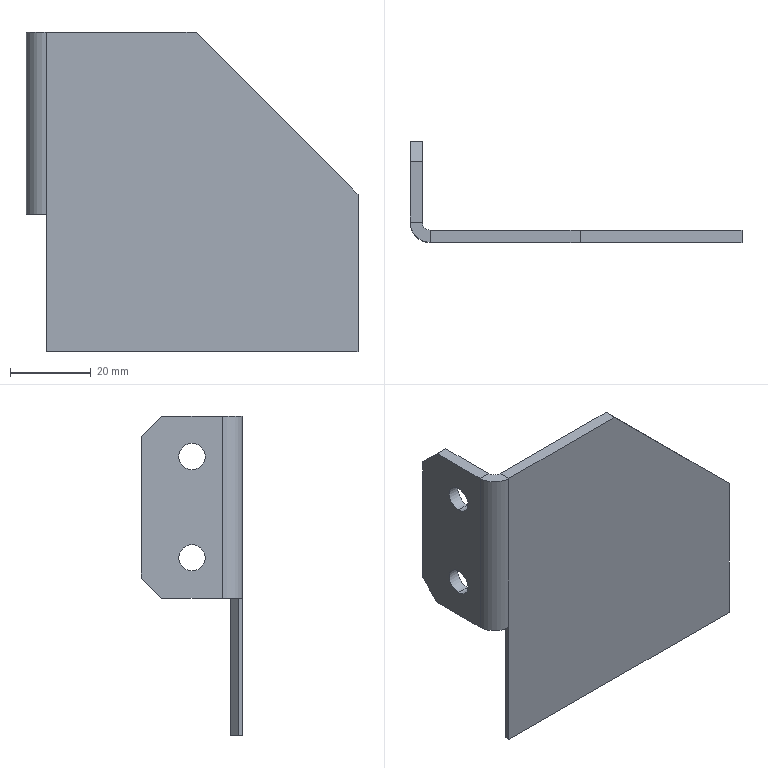Component | SolidWorks | OPW-05-033-1 | 1 solid | 22 faces | box 82 x 25 x 79 mm | volume 18949 mm3 | plane 16 | cylinder 6 | commonest cylinder face diameters 6.5 x4 4 x1 10 x1
STEP:
#1=COLOUR_RGB('',0.7922,0.8196,0.9333);
#2=FILL_AREA_STYLE_COLOUR('',#1);
#3=FILL_AREA_STYLE('',(#2));
#4=SURFACE_STYLE_FILL_AREA(#3);
#5=SURFACE_SIDE_STYLE('',(#4));
#6=SURFACE_STYLE_USAGE(.BOTH.,#5);
#7=PRESENTATION_STYLE_ASSIGNMENT((#6));
#8=CARTESIAN_POINT('',(1.775,9.035,0.9154));
#9=VERTEX_POINT('',#8);
#10=CARTESIAN_POINT('',(1.775,9.035,0.6594));
#11=VERTEX_POINT('',#10);
#12=CARTESIAN_POINT('',(1.775,9.035,0.7874));
#13=DIRECTION('',(1.,-0.,0.));
#14=DIRECTION('',(0.,1.,0.));
#15=AXIS2_PLACEMENT_3D('',#12,#13,#14);
#16=CIRCLE('',#15,0.128);
#17=EDGE_CURVE('',#9,#11,#16,.T.);
#18=ORIENTED_EDGE('',*,*,#17,.F.);
#19=CARTESIAN_POINT('',(1.894,9.035,0.9154));
#20=VERTEX_POINT('',#19);
#21=CARTESIAN_POINT('',(1.894,9.035,0.9154));
#22=DIRECTION('',(1.,0.,0.));
#23=VECTOR('',#22,39.37);
#24=LINE('',#21,#23);
#25=EDGE_CURVE('',#9,#20,#24,.T.);
#26=ORIENTED_EDGE('',*,*,#25,.T.);
#27=CARTESIAN_POINT('',(1.894,9.035,0.6594));
#28=VERTEX_POINT('',#27);
#29=CARTESIAN_POINT('',(1.894,9.035,0.7874));
#30=DIRECTION('',(1.,0.,0.));
#31=DIRECTION('',(0.,0.,-1.));
#32=AXIS2_PLACEMENT_3D('',#29,#30,#31);
#33=CIRCLE('',#32,0.128);
#34=EDGE_CURVE('',#20,#28,#33,.T.);
#35=ORIENTED_EDGE('',*,*,#34,.T.);
#36=CARTESIAN_POINT('',(1.894,9.035,0.6594));
#37=DIRECTION('',(1.,0.,0.));
#38=VECTOR('',#37,39.37);
#39=LINE('',#36,#38);
#40=EDGE_CURVE('',#11,#28,#39,.T.);
#41=ORIENTED_EDGE('',*,*,#40,.F.);
#42=EDGE_LOOP('',(#18,#26,#35,#41));
#43=FACE_OUTER_BOUND('',#42,.T.);
#44=CARTESIAN_POINT('',(1.894,9.035,0.7874));
#45=DIRECTION('',(1.,0.,0.));
#46=DIRECTION('',(0.,0.,-1.));
#47=AXIS2_PLACEMENT_3D('',#44,#45,#46);
#48=CYLINDRICAL_SURFACE('',#47,0.128);
#49=ADVANCED_FACE('',(#43),#48,.F.);
#50=CARTESIAN_POINT('',(1.775,9.035,-0.0689));
#51=VERTEX_POINT('',#50);
#52=CARTESIAN_POINT('',(1.775,9.035,-0.3248));
#53=VERTEX_POINT('',#52);
#54=CARTESIAN_POINT('',(1.775,9.035,-0.1969));
#55=DIRECTION('',(1.,-0.,0.));
#56=DIRECTION('',(0.,1.,0.));
#57=AXIS2_PLACEMENT_3D('',#54,#55,#56);
#58=CIRCLE('',#57,0.128);
#59=EDGE_CURVE('',#51,#53,#58,.T.);
#60=ORIENTED_EDGE('',*,*,#59,.F.);
#61=CARTESIAN_POINT('',(1.894,9.035,-0.0689));
#62=VERTEX_POINT('',#61);
#63=CARTESIAN_POINT('',(1.894,9.035,-0.0689));
#64=DIRECTION('',(1.,0.,0.));
#65=VECTOR('',#64,39.37);
#66=LINE('',#63,#65);
#67=EDGE_CURVE('',#51,#62,#66,.T.);
#68=ORIENTED_EDGE('',*,*,#67,.T.);
#69=CARTESIAN_POINT('',(1.894,9.035,-0.3248));
#70=VERTEX_POINT('',#69);
#71=CARTESIAN_POINT('',(1.894,9.035,-0.1969));
#72=DIRECTION('',(1.,0.,0.));
#73=DIRECTION('',(0.,0.,-1.));
#74=AXIS2_PLACEMENT_3D('',#71,#72,#73);
#75=CIRCLE('',#74,0.128);
#76=EDGE_CURVE('',#62,#70,#75,.T.);
#77=ORIENTED_EDGE('',*,*,#76,.T.);
#78=CARTESIAN_POINT('',(1.894,9.035,-0.3248));
#79=DIRECTION('',(1.,0.,0.));
#80=VECTOR('',#79,39.37);
#81=LINE('',#78,#80);
#82=EDGE_CURVE('',#53,#70,#81,.T.);
#83=ORIENTED_EDGE('',*,*,#82,.F.);
#84=EDGE_LOOP('',(#60,#68,#77,#83));
#85=FACE_OUTER_BOUND('',#84,.T.);
#86=CARTESIAN_POINT('',(1.894,9.035,-0.1969));
#87=DIRECTION('',(1.,0.,0.));
#88=DIRECTION('',(0.,0.,-1.));
#89=AXIS2_PLACEMENT_3D('',#86,#87,#88);
#90=CYLINDRICAL_SURFACE('',#89,0.128);
#91=ADVANCED_FACE('',(#85),#90,.F.);
#92=CARTESIAN_POINT('',(1.775,8.74,1.181));
#93=VERTEX_POINT('',#92);
#94=CARTESIAN_POINT('',(1.894,8.74,1.181));
#95=VERTEX_POINT('',#94);
#96=CARTESIAN_POINT('',(1.775,8.74,1.181));
#97=DIRECTION('',(1.,0.,0.));
#98=VECTOR('',#97,39.37);
#99=LINE('',#96,#98);
#100=EDGE_CURVE('',#93,#95,#99,.T.);
#101=ORIENTED_EDGE('',*,*,#100,.F.);
#102=CARTESIAN_POINT('',(1.972,8.543,1.181));
#103=VERTEX_POINT('',#102);
#104=CARTESIAN_POINT('',(1.972,8.74,1.181));
#105=DIRECTION('',(0.,0.,1.));
#106=DIRECTION('',(-1.,0.,0.));
#107=AXIS2_PLACEMENT_3D('',#104,#105,#106);
#108=CIRCLE('',#107,0.1969);
#109=EDGE_CURVE('',#93,#103,#108,.T.);
#110=ORIENTED_EDGE('',*,*,#109,.T.);
#111=CARTESIAN_POINT('',(1.972,8.661,1.181));
#112=VERTEX_POINT('',#111);
#113=CARTESIAN_POINT('',(1.972,8.661,1.181));
#114=DIRECTION('',(0.,-1.,0.));
#115=VECTOR('',#114,39.37);
#116=LINE('',#113,#115);
#117=EDGE_CURVE('',#112,#103,#116,.T.);
#118=ORIENTED_EDGE('',*,*,#117,.F.);
#119=CARTESIAN_POINT('',(1.972,8.74,1.181));
#120=DIRECTION('',(0.,0.,1.));
#121=DIRECTION('',(1.,0.,0.));
#122=AXIS2_PLACEMENT_3D('',#119,#120,#121);
#123=CIRCLE('',#122,0.07874);
#124=EDGE_CURVE('',#95,#112,#123,.T.);
#125=ORIENTED_EDGE('',*,*,#124,.F.);
#126=EDGE_LOOP('',(#101,#110,#118,#125));
#127=FACE_OUTER_BOUND('',#126,.T.);
#128=CARTESIAN_POINT('',(1.775,8.74,1.181));
#129=DIRECTION('',(0.,0.,1.));
#130=DIRECTION('',(1.,0.,0.));
#131=AXIS2_PLACEMENT_3D('',#128,#129,#130);
#132=PLANE('',#131);
#133=ADVANCED_FACE('',(#127),#132,.T.);
#134=CARTESIAN_POINT('',(1.894,9.331,1.181));
#135=VERTEX_POINT('',#134);
#136=CARTESIAN_POINT('',(1.894,9.528,1.181));
#137=DIRECTION('',(-0.,-1.,0.));
#138=VECTOR('',#137,39.37);
#139=LINE('',#136,#138);
#140=EDGE_CURVE('',#135,#95,#139,.T.);
#141=ORIENTED_EDGE('',*,*,#140,.F.);
#142=CARTESIAN_POINT('',(1.775,9.331,1.181));
#143=VERTEX_POINT('',#142);
#144=CARTESIAN_POINT('',(1.972,9.331,1.181));
#145=DIRECTION('',(-1.,0.,0.));
#146=VECTOR('',#145,39.37);
#147=LINE('',#144,#146);
#148=EDGE_CURVE('',#135,#143,#147,.T.);
#149=ORIENTED_EDGE('',*,*,#148,.T.);
#150=CARTESIAN_POINT('',(1.775,9.528,1.181));
#151=DIRECTION('',(-0.,-1.,0.));
#152=VECTOR('',#151,39.37);
#153=LINE('',#150,#152);
#154=EDGE_CURVE('',#143,#93,#153,.T.);
#155=ORIENTED_EDGE('',*,*,#154,.T.);
#156=ORIENTED_EDGE('',*,*,#100,.T.);
#157=EDGE_LOOP('',(#141,#149,#155,#156));
#158=FACE_OUTER_BOUND('',#157,.T.);
#159=CARTESIAN_POINT('',(1.972,8.661,1.181));
#160=DIRECTION('',(0.,0.,1.));
#161=DIRECTION('',(1.,0.,0.));
#162=AXIS2_PLACEMENT_3D('',#159,#160,#161);
#163=PLANE('',#162);
#164=ADVANCED_FACE('',(#158),#163,.T.);
#165=CARTESIAN_POINT('',(1.972,8.543,-1.929));
#166=VERTEX_POINT('',#165);
#167=CARTESIAN_POINT('',(1.972,8.583,-1.929));
#168=VERTEX_POINT('',#167);
#169=CARTESIAN_POINT('',(1.972,8.543,-1.929));
#170=DIRECTION('',(0.,1.,0.));
#171=VECTOR('',#170,39.37);
#172=LINE('',#169,#171);
#173=EDGE_CURVE('',#166,#168,#172,.T.);
#174=ORIENTED_EDGE('',*,*,#173,.T.);
#175=CARTESIAN_POINT('',(2.051,8.661,-1.929));
#176=VERTEX_POINT('',#175);
#177=CARTESIAN_POINT('',(2.012,8.622,-1.929));
#178=DIRECTION('',(0.7071,0.7071,0.));
#179=VECTOR('',#178,39.37);
#180=LINE('',#177,#179);
#181=EDGE_CURVE('',#168,#176,#180,.T.);
#182=ORIENTED_EDGE('',*,*,#181,.T.);
#183=CARTESIAN_POINT('',(5.004,8.661,-1.929));
#184=VERTEX_POINT('',#183);
#185=CARTESIAN_POINT('',(1.775,8.661,-1.929));
#186=DIRECTION('',(1.,0.,0.));
#187=VECTOR('',#186,39.37);
#188=LINE('',#185,#187);
#189=EDGE_CURVE('',#176,#184,#188,.T.);
#190=ORIENTED_EDGE('',*,*,#189,.T.);
#191=CARTESIAN_POINT('',(5.004,8.543,-1.929));
#192=VERTEX_POINT('',#191);
#193=CARTESIAN_POINT('',(5.004,8.661,-1.929));
#194=DIRECTION('',(0.,-1.,0.));
#195=VECTOR('',#194,39.37);
#196=LINE('',#193,#195);
#197=EDGE_CURVE('',#184,#192,#196,.T.);
#198=ORIENTED_EDGE('',*,*,#197,.T.);
#199=CARTESIAN_POINT('',(1.775,8.543,-1.929));
#200=DIRECTION('',(1.,0.,0.));
#201=VECTOR('',#200,39.37);
#202=LINE('',#199,#201);
#203=EDGE_CURVE('',#166,#192,#202,.T.);
#204=ORIENTED_EDGE('',*,*,#203,.F.);
#205=EDGE_LOOP('',(#174,#182,#190,#198,#204));
#206=FACE_OUTER_BOUND('',#205,.T.);
#207=CARTESIAN_POINT('',(1.894,8.74,-1.929));
#208=DIRECTION('',(0.,0.,-1.));
#209=DIRECTION('',(-1.,0.,0.));
#210=AXIS2_PLACEMENT_3D('',#207,#208,#209);
#211=PLANE('',#210);
#212=ADVANCED_FACE('',(#206),#211,.T.);
#213=CARTESIAN_POINT('',(5.004,8.543,-0.3937));
#214=VERTEX_POINT('',#213);
#215=CARTESIAN_POINT('',(5.004,8.543,1.181));
#216=DIRECTION('',(0.,0.,-1.));
#217=VECTOR('',#216,39.37);
#218=LINE('',#215,#217);
#219=EDGE_CURVE('',#214,#192,#218,.T.);
#220=ORIENTED_EDGE('',*,*,#219,.F.);
#221=CARTESIAN_POINT('',(3.429,8.543,1.181));
#222=VERTEX_POINT('',#221);
#223=CARTESIAN_POINT('',(5.004,8.543,-0.3937));
#224=DIRECTION('',(-0.7071,0.,0.7071));
#225=VECTOR('',#224,39.37);
#226=LINE('',#223,#225);
#227=EDGE_CURVE('',#214,#222,#226,.T.);
#228=ORIENTED_EDGE('',*,*,#227,.T.);
#229=CARTESIAN_POINT('',(1.775,8.543,1.181));
#230=DIRECTION('',(1.,0.,0.));
#231=VECTOR('',#230,39.37);
#232=LINE('',#229,#231);
#233=EDGE_CURVE('',#103,#222,#232,.T.);
#234=ORIENTED_EDGE('',*,*,#233,.F.);
#235=CARTESIAN_POINT('',(1.972,8.543,-0.5906));
#236=VERTEX_POINT('',#235);
#237=CARTESIAN_POINT('',(1.972,8.543,1.181));
#238=DIRECTION('',(0.,0.,-1.));
#239=VECTOR('',#238,39.37);
#240=LINE('',#237,#239);
#241=EDGE_CURVE('',#103,#236,#240,.T.);
#242=ORIENTED_EDGE('',*,*,#241,.T.);
#243=CARTESIAN_POINT('',(1.972,8.543,-1.929));
#244=DIRECTION('',(-0.,0.,-1.));
#245=VECTOR('',#244,39.37);
#246=LINE('',#243,#245);
#247=EDGE_CURVE('',#236,#166,#246,.T.);
#248=ORIENTED_EDGE('',*,*,#247,.T.);
#249=ORIENTED_EDGE('',*,*,#203,.T.);
#250=EDGE_LOOP('',(#220,#228,#234,#242,#248,#249));
#251=FACE_OUTER_BOUND('',#250,.T.);
#252=CARTESIAN_POINT('',(1.775,8.543,1.181));
#253=DIRECTION('',(0.,1.,0.));
#254=DIRECTION('',(0.,0.,1.));
#255=AXIS2_PLACEMENT_3D('',#252,#253,#254);
#256=PLANE('',#255);
#257=ADVANCED_FACE('',(#251),#256,.F.);
#258=CARTESIAN_POINT('',(5.004,8.661,-0.3937));
#259=VERTEX_POINT('',#258);
#260=CARTESIAN_POINT('',(5.004,8.661,1.181));
#261=DIRECTION('',(0.,0.,-1.));
#262=VECTOR('',#261,39.37);
#263=LINE('',#260,#262);
#264=EDGE_CURVE('',#259,#184,#263,.T.);
#265=ORIENTED_EDGE('',*,*,#264,.F.);
#266=CARTESIAN_POINT('',(5.004,8.661,-0.3937));
#267=DIRECTION('',(0.,-1.,0.));
#268=VECTOR('',#267,39.37);
#269=LINE('',#266,#268);
#270=EDGE_CURVE('',#259,#214,#269,.T.);
#271=ORIENTED_EDGE('',*,*,#270,.T.);
#272=ORIENTED_EDGE('',*,*,#219,.T.);
#273=ORIENTED_EDGE('',*,*,#197,.F.);
#274=EDGE_LOOP('',(#265,#271,#272,#273));
#275=FACE_OUTER_BOUND('',#274,.T.);
#276=CARTESIAN_POINT('',(5.004,8.661,1.181));
#277=DIRECTION('',(1.,0.,0.));
#278=DIRECTION('',(0.,0.,-1.));
#279=AXIS2_PLACEMENT_3D('',#276,#277,#278);
#280=PLANE('',#279);
#281=ADVANCED_FACE('',(#275),#280,.T.);
#282=CARTESIAN_POINT('',(3.429,8.661,1.181));
#283=VERTEX_POINT('',#282);
#284=CARTESIAN_POINT('',(1.775,8.661,1.181));
#285=DIRECTION('',(1.,0.,0.));
#286=VECTOR('',#285,39.37);
#287=LINE('',#284,#286);
#288=EDGE_CURVE('',#112,#283,#287,.T.);
#289=ORIENTED_EDGE('',*,*,#288,.T.);
#290=CARTESIAN_POINT('',(2.602,8.661,2.008));
#291=DIRECTION('',(0.7071,0.,-0.7071));
#292=VECTOR('',#291,39.37);
#293=LINE('',#290,#292);
#294=EDGE_CURVE('',#283,#259,#293,.T.);
#295=ORIENTED_EDGE('',*,*,#294,.T.);
#296=ORIENTED_EDGE('',*,*,#264,.T.);
#297=ORIENTED_EDGE('',*,*,#189,.F.);
#298=CARTESIAN_POINT('',(2.051,8.661,-0.5906));
#299=VERTEX_POINT('',#298);
#300=CARTESIAN_POINT('',(2.051,8.661,-0.5906));
#301=DIRECTION('',(0.,0.,1.));
#302=VECTOR('',#301,39.37);
#303=LINE('',#300,#302);
#304=EDGE_CURVE('',#176,#299,#303,.T.);
#305=ORIENTED_EDGE('',*,*,#304,.T.);
#306=CARTESIAN_POINT('',(1.972,8.661,-0.5906));
#307=VERTEX_POINT('',#306);
#308=CARTESIAN_POINT('',(1.775,8.661,-0.5906));
#309=DIRECTION('',(-1.,0.,0.));
#310=VECTOR('',#309,39.37);
#311=LINE('',#308,#310);
#312=EDGE_CURVE('',#299,#307,#311,.T.);
#313=ORIENTED_EDGE('',*,*,#312,.T.);
#314=CARTESIAN_POINT('',(1.972,8.661,1.181));
#315=DIRECTION('',(0.,0.,-1.));
#316=VECTOR('',#315,39.37);
#317=LINE('',#314,#316);
#318=EDGE_CURVE('',#112,#307,#317,.T.);
#319=ORIENTED_EDGE('',*,*,#318,.F.);
#320=EDGE_LOOP('',(#289,#295,#296,#297,#305,#313,#319));
#321=FACE_OUTER_BOUND('',#320,.T.);
#322=CARTESIAN_POINT('',(1.775,8.661,1.181));
#323=DIRECTION('',(0.,1.,0.));
#324=DIRECTION('',(0.,0.,1.));
#325=AXIS2_PLACEMENT_3D('',#322,#323,#324);
#326=PLANE('',#325);
#327=ADVANCED_FACE('',(#321),#326,.T.);
#328=CARTESIAN_POINT('',(1.894,8.74,-0.5906));
#329=VERTEX_POINT('',#328);
#330=CARTESIAN_POINT('',(1.972,8.74,-0.5906));
#331=DIRECTION('',(0.,0.,1.));
#332=DIRECTION('',(1.,0.,0.));
#333=AXIS2_PLACEMENT_3D('',#330,#331,#332);
#334=CIRCLE('',#333,0.07874);
#335=EDGE_CURVE('',#329,#307,#334,.T.);
#336=ORIENTED_EDGE('',*,*,#335,.F.);
#337=CARTESIAN_POINT('',(1.894,8.74,1.181));
#338=DIRECTION('',(0.,0.,-1.));
#339=VECTOR('',#338,39.37);
#340=LINE('',#337,#339);
#341=EDGE_CURVE('',#95,#329,#340,.T.);
#342=ORIENTED_EDGE('',*,*,#341,.F.);
#343=ORIENTED_EDGE('',*,*,#124,.T.);
#344=ORIENTED_EDGE('',*,*,#318,.T.);
#345=EDGE_LOOP('',(#336,#342,#343,#344));
#346=FACE_OUTER_BOUND('',#345,.T.);
#347=CARTESIAN_POINT('',(1.972,8.74,1.181));
#348=DIRECTION('',(0.,0.,-1.));
#349=DIRECTION('',(-1.,0.,0.));
#350=AXIS2_PLACEMENT_3D('',#347,#348,#349);
#351=CYLINDRICAL_SURFACE('',#350,0.07874);
#352=ADVANCED_FACE('',(#346),#351,.F.);
#353=CARTESIAN_POINT('',(1.894,9.331,-0.5906));
#354=VERTEX_POINT('',#353);
#355=CARTESIAN_POINT('',(1.894,9.528,-0.5906));
#356=DIRECTION('',(-0.,-1.,0.));
#357=VECTOR('',#356,39.37);
#358=LINE('',#355,#357);
#359=EDGE_CURVE('',#354,#329,#358,.T.);
#360=ORIENTED_EDGE('',*,*,#359,.F.);
#361=CARTESIAN_POINT('',(1.894,9.528,-0.3937));
#362=VERTEX_POINT('',#361);
#363=CARTESIAN_POINT('',(1.894,10.315,0.3937));
#364=DIRECTION('',(0.,0.7071,0.7071));
#365=VECTOR('',#364,39.37);
#366=LINE('',#363,#365);
#367=EDGE_CURVE('',#354,#362,#366,.T.);
#368=ORIENTED_EDGE('',*,*,#367,.T.);
#369=CARTESIAN_POINT('',(1.894,9.528,0.9843));
#370=VERTEX_POINT('',#369);
#371=CARTESIAN_POINT('',(1.894,9.528,1.181));
#372=DIRECTION('',(0.,0.,-1.));
#373=VECTOR('',#372,39.37);
#374=LINE('',#371,#373);
#375=EDGE_CURVE('',#370,#362,#374,.T.);
#376=ORIENTED_EDGE('',*,*,#375,.F.);
#377=CARTESIAN_POINT('',(1.894,9.429,1.083));
#378=DIRECTION('',(-0.,-0.7071,0.7071));
#379=VECTOR('',#378,39.37);
#380=LINE('',#377,#379);
#381=EDGE_CURVE('',#370,#135,#380,.T.);
#382=ORIENTED_EDGE('',*,*,#381,.T.);
#383=ORIENTED_EDGE('',*,*,#140,.T.);
#384=ORIENTED_EDGE('',*,*,#341,.T.);
#385=EDGE_LOOP('',(#360,#368,#376,#382,#383,#384));
#386=FACE_OUTER_BOUND('',#385,.T.);
#387=CARTESIAN_POINT('',(1.894,9.035,0.7874));
#388=DIRECTION('',(1.,0.,0.));
#389=DIRECTION('',(0.,0.,-1.));
#390=AXIS2_PLACEMENT_3D('',#387,#388,#389);
#391=CIRCLE('',#390,0.128);
#392=EDGE_CURVE('',#28,#20,#391,.T.);
#393=ORIENTED_EDGE('',*,*,#392,.F.);
#394=ORIENTED_EDGE('',*,*,#34,.F.);
#395=EDGE_LOOP('',(#393,#394));
#396=FACE_BOUND('',#395,.T.);
#397=CARTESIAN_POINT('',(1.894,9.035,-0.1969));
#398=DIRECTION('',(1.,0.,0.));
#399=DIRECTION('',(0.,0.,-1.));
#400=AXIS2_PLACEMENT_3D('',#397,#398,#399);
#401=CIRCLE('',#400,0.128);
#402=EDGE_CURVE('',#70,#62,#401,.T.);
#403=ORIENTED_EDGE('',*,*,#402,.F.);
#404=ORIENTED_EDGE('',*,*,#76,.F.);
#405=EDGE_LOOP('',(#403,#404));
#406=FACE_BOUND('',#405,.T.);
#407=CARTESIAN_POINT('',(1.894,9.528,1.181));
#408=DIRECTION('',(1.,-0.,0.));
#409=DIRECTION('',(0.,1.,0.));
#410=AXIS2_PLACEMENT_3D('',#407,#408,#409);
#411=PLANE('',#410);
#412=ADVANCED_FACE('',(#386,#396,#406),#411,.T.);
#413=ORIENTED_EDGE('',*,*,#375,.T.);
#414=CARTESIAN_POINT('',(1.775,9.528,-0.3937));
#415=VERTEX_POINT('',#414);
#416=CARTESIAN_POINT('',(1.775,9.528,-0.3937));
#417=DIRECTION('',(-1.,0.,0.));
#418=VECTOR('',#417,39.37);
#419=LINE('',#416,#418);
#420=EDGE_CURVE('',#362,#415,#419,.T.);
#421=ORIENTED_EDGE('',*,*,#420,.T.);
#422=CARTESIAN_POINT('',(1.775,9.528,0.9843));
#423=VERTEX_POINT('',#422);
#424=CARTESIAN_POINT('',(1.775,9.528,1.181));
#425=DIRECTION('',(0.,0.,-1.));
#426=VECTOR('',#425,39.37);
#427=LINE('',#424,#426);
#428=EDGE_CURVE('',#423,#415,#427,.T.);
#429=ORIENTED_EDGE('',*,*,#428,.F.);
#430=CARTESIAN_POINT('',(1.775,9.528,0.9843));
#431=DIRECTION('',(1.,0.,0.));
#432=VECTOR('',#431,39.37);
#433=LINE('',#430,#432);
#434=EDGE_CURVE('',#423,#370,#433,.T.);
#435=ORIENTED_EDGE('',*,*,#434,.T.);
#436=EDGE_LOOP('',(#413,#421,#429,#435));
#437=FACE_OUTER_BOUND('',#436,.T.);
#438=CARTESIAN_POINT('',(1.775,9.528,1.181));
#439=DIRECTION('',(0.,1.,0.));
#440=DIRECTION('',(0.,0.,1.));
#441=AXIS2_PLACEMENT_3D('',#438,#439,#440);
#442=PLANE('',#441);
#443=ADVANCED_FACE('',(#437),#442,.T.);
#444=CARTESIAN_POINT('',(1.775,9.035,0.7874));
#445=DIRECTION('',(1.,-0.,0.));
#446=DIRECTION('',(0.,1.,0.));
#447=AXIS2_PLACEMENT_3D('',#444,#445,#446);
#448=CIRCLE('',#447,0.128);
#449=EDGE_CURVE('',#11,#9,#448,.T.);
#450=ORIENTED_EDGE('',*,*,#449,.T.);
#451=ORIENTED_EDGE('',*,*,#17,.T.);
#452=EDGE_LOOP('',(#450,#451));
#453=FACE_BOUND('',#452,.T.);
#454=CARTESIAN_POINT('',(1.775,9.035,-0.1969));
#455=DIRECTION('',(1.,-0.,0.));
#456=DIRECTION('',(0.,1.,0.));
#457=AXIS2_PLACEMENT_3D('',#454,#455,#456);
#458=CIRCLE('',#457,0.128);
#459=EDGE_CURVE('',#53,#51,#458,.T.);
#460=ORIENTED_EDGE('',*,*,#459,.T.);
#461=ORIENTED_EDGE('',*,*,#59,.T.);
#462=EDGE_LOOP('',(#460,#461));
#463=FACE_BOUND('',#462,.T.);
#464=ORIENTED_EDGE('',*,*,#428,.T.);
#465=CARTESIAN_POINT('',(1.775,9.331,-0.5906));
#466=VERTEX_POINT('',#465);
#467=CARTESIAN_POINT('',(1.775,9.331,-0.5906));
#468=DIRECTION('',(-0.,-0.7071,-0.7071));
#469=VECTOR('',#468,39.37);
#470=LINE('',#467,#469);
#471=EDGE_CURVE('',#415,#466,#470,.T.);
#472=ORIENTED_EDGE('',*,*,#471,.T.);
#473=CARTESIAN_POINT('',(1.775,8.74,-0.5906));
#474=VERTEX_POINT('',#473);
#475=CARTESIAN_POINT('',(1.775,8.543,-0.5906));
#476=DIRECTION('',(0.,1.,0.));
#477=VECTOR('',#476,39.37);
#478=LINE('',#475,#477);
#479=EDGE_CURVE('',#474,#466,#478,.T.);
#480=ORIENTED_EDGE('',*,*,#479,.F.);
#481=CARTESIAN_POINT('',(1.775,8.74,1.181));
#482=DIRECTION('',(0.,0.,-1.));
#483=VECTOR('',#482,39.37);
#484=LINE('',#481,#483);
#485=EDGE_CURVE('',#93,#474,#484,.T.);
#486=ORIENTED_EDGE('',*,*,#485,.F.);
#487=ORIENTED_EDGE('',*,*,#154,.F.);
#488=CARTESIAN_POINT('',(1.775,9.528,0.9843));
#489=DIRECTION('',(0.,0.7071,-0.7071));
#490=VECTOR('',#489,39.37);
#491=LINE('',#488,#490);
#492=EDGE_CURVE('',#143,#423,#491,.T.);
#493=ORIENTED_EDGE('',*,*,#492,.T.);
#494=EDGE_LOOP('',(#464,#472,#480,#486,#487,#493));
#495=FACE_OUTER_BOUND('',#494,.T.);
#496=CARTESIAN_POINT('',(1.775,9.528,1.181));
#497=DIRECTION('',(1.,-0.,0.));
#498=DIRECTION('',(0.,1.,0.));
#499=AXIS2_PLACEMENT_3D('',#496,#497,#498);
#500=PLANE('',#499);
#501=ADVANCED_FACE('',(#453,#463,#495),#500,.F.);
#502=ORIENTED_EDGE('',*,*,#485,.T.);
#503=CARTESIAN_POINT('',(1.972,8.74,-0.5906));
#504=DIRECTION('',(0.,0.,1.));
#505=DIRECTION('',(1.,0.,0.));
#506=AXIS2_PLACEMENT_3D('',#503,#504,#505);
#507=CIRCLE('',#506,0.1969);
#508=EDGE_CURVE('',#474,#236,#507,.T.);
#509=ORIENTED_EDGE('',*,*,#508,.T.);
#510=ORIENTED_EDGE('',*,*,#241,.F.);
#511=ORIENTED_EDGE('',*,*,#109,.F.);
#512=EDGE_LOOP('',(#502,#509,#510,#511));
#513=FACE_OUTER_BOUND('',#512,.T.);
#514=CARTESIAN_POINT('',(1.972,8.74,1.181));
#515=DIRECTION('',(0.,0.,-1.));
#516=DIRECTION('',(-1.,0.,0.));
#517=AXIS2_PLACEMENT_3D('',#514,#515,#516);
#518=CYLINDRICAL_SURFACE('',#517,0.1969);
#519=ADVANCED_FACE('',(#513),#518,.T.);
#520=ORIENTED_EDGE('',*,*,#233,.T.);
#521=CARTESIAN_POINT('',(3.429,8.74,1.181));
#522=DIRECTION('',(0.,1.,0.));
#523=VECTOR('',#522,39.37);
#524=LINE('',#521,#523);
#525=EDGE_CURVE('',#222,#283,#524,.T.);
#526=ORIENTED_EDGE('',*,*,#525,.T.);
#527=ORIENTED_EDGE('',*,*,#288,.F.);
#528=ORIENTED_EDGE('',*,*,#117,.T.);
#529=EDGE_LOOP('',(#520,#526,#527,#528));
#530=FACE_OUTER_BOUND('',#529,.T.);
#531=CARTESIAN_POINT('',(1.972,8.74,1.181));
#532=DIRECTION('',(0.,0.,1.));
#533=DIRECTION('',(1.,0.,0.));
#534=AXIS2_PLACEMENT_3D('',#531,#532,#533);
#535=PLANE('',#534);
#536=ADVANCED_FACE('',(#530),#535,.T.);
#537=ORIENTED_EDGE('',*,*,#67,.F.);
#538=ORIENTED_EDGE('',*,*,#459,.F.);
#539=ORIENTED_EDGE('',*,*,#82,.T.);
#540=ORIENTED_EDGE('',*,*,#402,.T.);
#541=EDGE_LOOP('',(#537,#538,#539,#540));
#542=FACE_OUTER_BOUND('',#541,.T.);
#543=CARTESIAN_POINT('',(1.894,9.035,-0.1969));
#544=DIRECTION('',(1.,0.,0.));
#545=DIRECTION('',(0.,0.,-1.));
#546=AXIS2_PLACEMENT_3D('',#543,#544,#545);
#547=CYLINDRICAL_SURFACE('',#546,0.128);
#548=ADVANCED_FACE('',(#542),#547,.F.);
#549=ORIENTED_EDGE('',*,*,#25,.F.);
#550=ORIENTED_EDGE('',*,*,#449,.F.);
#551=ORIENTED_EDGE('',*,*,#40,.T.);
#552=ORIENTED_EDGE('',*,*,#392,.T.);
#553=EDGE_LOOP('',(#549,#550,#551,#552));
#554=FACE_OUTER_BOUND('',#553,.T.);
#555=CARTESIAN_POINT('',(1.894,9.035,0.7874));
#556=DIRECTION('',(1.,0.,0.));
#557=DIRECTION('',(0.,0.,-1.));
#558=AXIS2_PLACEMENT_3D('',#555,#556,#557);
#559=CYLINDRICAL_SURFACE('',#558,0.128);
#560=ADVANCED_FACE('',(#554),#559,.F.);
#561=ORIENTED_EDGE('',*,*,#479,.T.);
#562=CARTESIAN_POINT('',(1.894,9.331,-0.5906));
#563=DIRECTION('',(1.,0.,0.));
#564=VECTOR('',#563,39.37);
#565=LINE('',#562,#564);
#566=EDGE_CURVE('',#466,#354,#565,.T.);
#567=ORIENTED_EDGE('',*,*,#566,.T.);
#568=ORIENTED_EDGE('',*,*,#359,.T.);
#569=ORIENTED_EDGE('',*,*,#335,.T.);
#570=ORIENTED_EDGE('',*,*,#312,.F.);
#571=CARTESIAN_POINT('',(1.972,8.583,-0.5906));
#572=VERTEX_POINT('',#571);
#573=CARTESIAN_POINT('',(1.854,8.465,-0.5906));
#574=DIRECTION('',(-0.7071,-0.7071,0.));
#575=VECTOR('',#574,39.37);
#576=LINE('',#573,#575);
#577=EDGE_CURVE('',#299,#572,#576,.T.);
#578=ORIENTED_EDGE('',*,*,#577,.T.);
#579=CARTESIAN_POINT('',(1.972,8.543,-0.5906));
#580=DIRECTION('',(0.,1.,0.));
#581=VECTOR('',#580,39.37);
#582=LINE('',#579,#581);
#583=EDGE_CURVE('',#236,#572,#582,.T.);
#584=ORIENTED_EDGE('',*,*,#583,.F.);
#585=ORIENTED_EDGE('',*,*,#508,.F.);
#586=EDGE_LOOP('',(#561,#567,#568,#569,#570,#578,#584,#585));
#587=FACE_OUTER_BOUND('',#586,.T.);
#588=CARTESIAN_POINT('',(1.775,8.543,-0.5906));
#589=DIRECTION('',(0.,0.,1.));
#590=DIRECTION('',(1.,0.,0.));
#591=AXIS2_PLACEMENT_3D('',#588,#589,#590);
#592=PLANE('',#591);
#593=ADVANCED_FACE('',(#587),#592,.F.);
#594=ORIENTED_EDGE('',*,*,#583,.T.);
#595=CARTESIAN_POINT('',(1.972,8.583,-1.929));
#596=DIRECTION('',(-0.,0.,-1.));
#597=VECTOR('',#596,39.37);
#598=LINE('',#595,#597);
#599=EDGE_CURVE('',#572,#168,#598,.T.);
#600=ORIENTED_EDGE('',*,*,#599,.T.);
#601=ORIENTED_EDGE('',*,*,#173,.F.);
#602=ORIENTED_EDGE('',*,*,#247,.F.);
#603=EDGE_LOOP('',(#594,#600,#601,#602));
#604=FACE_OUTER_BOUND('',#603,.T.);
#605=CARTESIAN_POINT('',(1.972,8.543,-1.929));
#606=DIRECTION('',(1.,0.,-0.));
#607=DIRECTION('',(-0.,0.,-1.));
#608=AXIS2_PLACEMENT_3D('',#605,#606,#607);
#609=PLANE('',#608);
#610=ADVANCED_FACE('',(#604),#609,.F.);
#611=ORIENTED_EDGE('',*,*,#577,.F.);
#612=ORIENTED_EDGE('',*,*,#304,.F.);
#613=ORIENTED_EDGE('',*,*,#181,.F.);
#614=ORIENTED_EDGE('',*,*,#599,.F.);
#615=EDGE_LOOP('',(#611,#612,#613,#614));
#616=FACE_OUTER_BOUND('',#615,.T.);
#617=CARTESIAN_POINT('',(1.972,8.583,-1.929));
#618=DIRECTION('',(-0.7071,0.7071,0.));
#619=DIRECTION('',(-0.7071,-0.7071,0.));
#620=AXIS2_PLACEMENT_3D('',#617,#618,#619);
#621=PLANE('',#620);
#622=ADVANCED_FACE('',(#616),#621,.T.);
#623=ORIENTED_EDGE('',*,*,#294,.F.);
#624=ORIENTED_EDGE('',*,*,#525,.F.);
#625=ORIENTED_EDGE('',*,*,#227,.F.);
#626=ORIENTED_EDGE('',*,*,#270,.F.);
#627=EDGE_LOOP('',(#623,#624,#625,#626));
#628=FACE_OUTER_BOUND('',#627,.T.);
#629=CARTESIAN_POINT('',(5.004,8.661,-0.3937));
#630=DIRECTION('',(-0.7071,0.,-0.7071));
#631=DIRECTION('',(-0.7071,0.,0.7071));
#632=AXIS2_PLACEMENT_3D('',#629,#630,#631);
#633=PLANE('',#632);
#634=ADVANCED_FACE('',(#628),#633,.F.);
#635=ORIENTED_EDGE('',*,*,#471,.F.);
#636=ORIENTED_EDGE('',*,*,#420,.F.);
#637=ORIENTED_EDGE('',*,*,#367,.F.);
#638=ORIENTED_EDGE('',*,*,#566,.F.);
#639=EDGE_LOOP('',(#635,#636,#637,#638));
#640=FACE_OUTER_BOUND('',#639,.T.);
#641=CARTESIAN_POINT('',(1.775,9.331,-0.5906));
#642=DIRECTION('',(0.,0.7071,-0.7071));
#643=DIRECTION('',(0.,0.7071,0.7071));
#644=AXIS2_PLACEMENT_3D('',#641,#642,#643);
#645=PLANE('',#644);
#646=ADVANCED_FACE('',(#640),#645,.T.);
#647=ORIENTED_EDGE('',*,*,#492,.F.);
#648=ORIENTED_EDGE('',*,*,#148,.F.);
#649=ORIENTED_EDGE('',*,*,#381,.F.);
#650=ORIENTED_EDGE('',*,*,#434,.F.);
#651=EDGE_LOOP('',(#647,#648,#649,#650));
#652=FACE_OUTER_BOUND('',#651,.T.);
#653=CARTESIAN_POINT('',(1.775,9.528,0.9843));
#654=DIRECTION('',(0.,-0.7071,-0.7071));
#655=DIRECTION('',(0.,0.7071,-0.7071));
#656=AXIS2_PLACEMENT_3D('',#653,#654,#655);
#657=PLANE('',#656);
#658=ADVANCED_FACE('',(#652),#657,.F.);
#659=CLOSED_SHELL('',(#49,#91,#133,#164,#212,#257,#281,#327,#352,#412,#443,#501,#519,#536,#548,#560,#593,#610,#622,#634,#646,#658));
#660=MANIFOLD_SOLID_BREP('',#659);
#661=STYLED_ITEM('',(#7),#660);
#662=(LENGTH_UNIT()NAMED_UNIT(*)SI_UNIT($,.METRE.));
#663=LENGTH_MEASURE_WITH_UNIT(LENGTH_MEASURE(0.0254),#662);
#664=DIMENSIONAL_EXPONENTS(1.,0.,0.,0.,0.,0.,0.);
#665=(CONVERSION_BASED_UNIT('',#663)LENGTH_UNIT()NAMED_UNIT(#664));
#666=UNCERTAINTY_MEASURE_WITH_UNIT(LENGTH_MEASURE(0.00001),#665,'','');
#667=(NAMED_UNIT(*)PLANE_ANGLE_UNIT()SI_UNIT($,.RADIAN.));
#668=(NAMED_UNIT(*)SI_UNIT($,.STERADIAN.)SOLID_ANGLE_UNIT());
#669=(GEOMETRIC_REPRESENTATION_CONTEXT(3)GLOBAL_UNCERTAINTY_ASSIGNED_CONTEXT((#666))GLOBAL_UNIT_ASSIGNED_CONTEXT((#665,#667,#668))REPRESENTATION_CONTEXT('',''));
#670=MECHANICAL_DESIGN_GEOMETRIC_PRESENTATION_REPRESENTATION('',(#661),#669);
#671=PRESENTATION_LAYER_ASSIGNMENT('','',(#661));
#672=CARTESIAN_POINT('',(0.,0.,0.));
#673=DIRECTION('',(0.,0.,1.));
#674=DIRECTION('',(1.,0.,0.));
#675=AXIS2_PLACEMENT_3D('',#672,#673,#674);
#676=(LENGTH_UNIT()NAMED_UNIT(*)SI_UNIT($,.METRE.));
#677=LENGTH_MEASURE_WITH_UNIT(LENGTH_MEASURE(0.0254),#676);
#678=DIMENSIONAL_EXPONENTS(1.,0.,0.,0.,0.,0.,0.);
#679=(CONVERSION_BASED_UNIT('',#677)LENGTH_UNIT()NAMED_UNIT(#678));
#680=UNCERTAINTY_MEASURE_WITH_UNIT(LENGTH_MEASURE(0.00001),#679,'','');
#681=(NAMED_UNIT(*)PLANE_ANGLE_UNIT()SI_UNIT($,.RADIAN.));
#682=(NAMED_UNIT(*)SI_UNIT($,.STERADIAN.)SOLID_ANGLE_UNIT());
#683=(GEOMETRIC_REPRESENTATION_CONTEXT(3)GLOBAL_UNCERTAINTY_ASSIGNED_CONTEXT((#680))GLOBAL_UNIT_ASSIGNED_CONTEXT((#679,#681,#682))REPRESENTATION_CONTEXT('',''));
#684=ADVANCED_BREP_SHAPE_REPRESENTATION('',(#660,#675),#683);